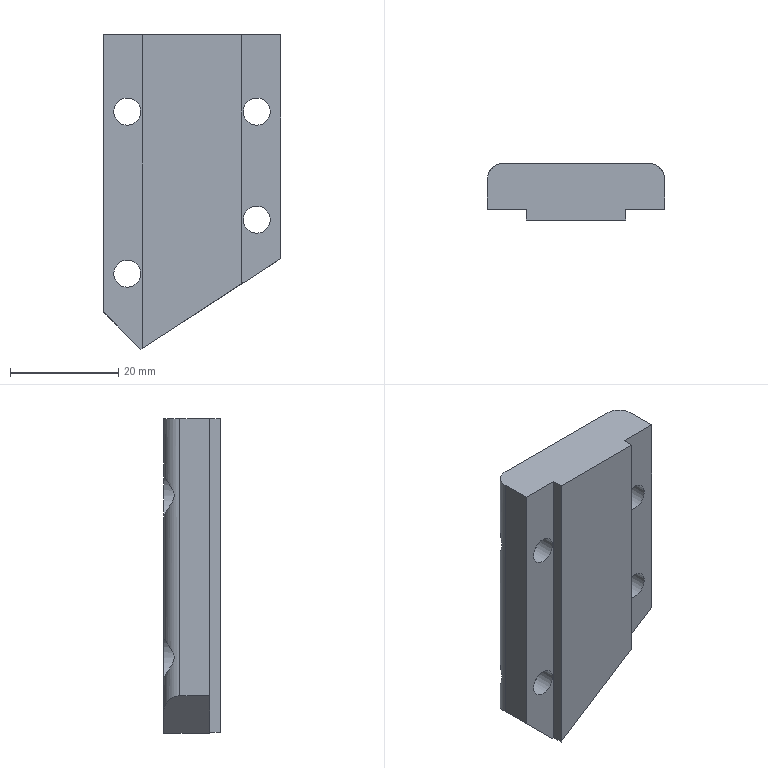Component | NX | YMSR_PET_P02 | 1 solid | 25 faces | volume 14581 mm3 | plane 15 | cylinder 10 | commonest cylinder face diameters 5 x4 8.5 x4 6 x2